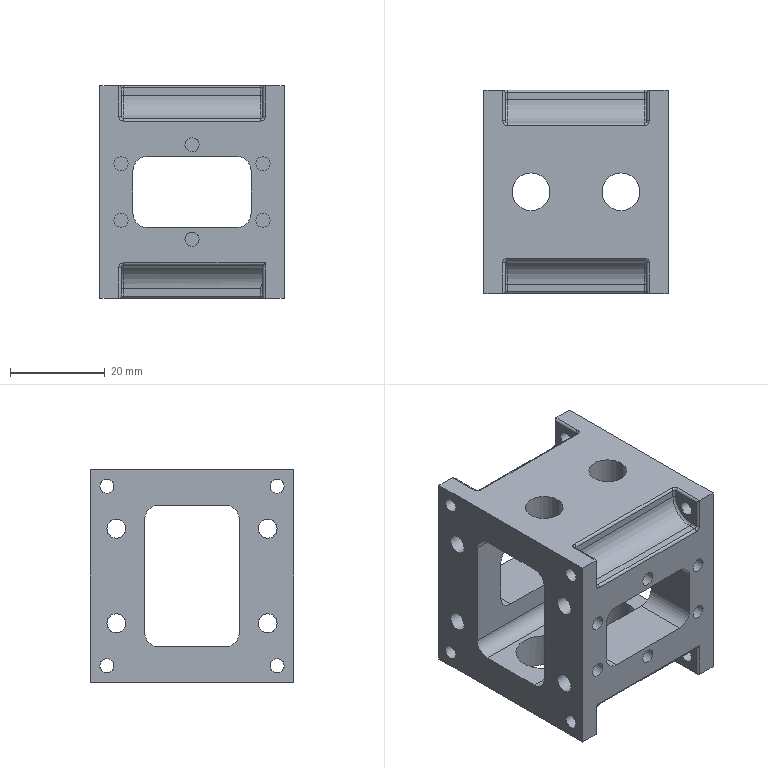Component | NX | 05A__27 | 1 solid | 150 faces | volume 33429 mm3 | cylinder 85 | plane 46 | torus 19 | commonest cylinder face diameters 1 x37 3 x24 6 x12 4 x4 10 x4 8 x2 12 x2